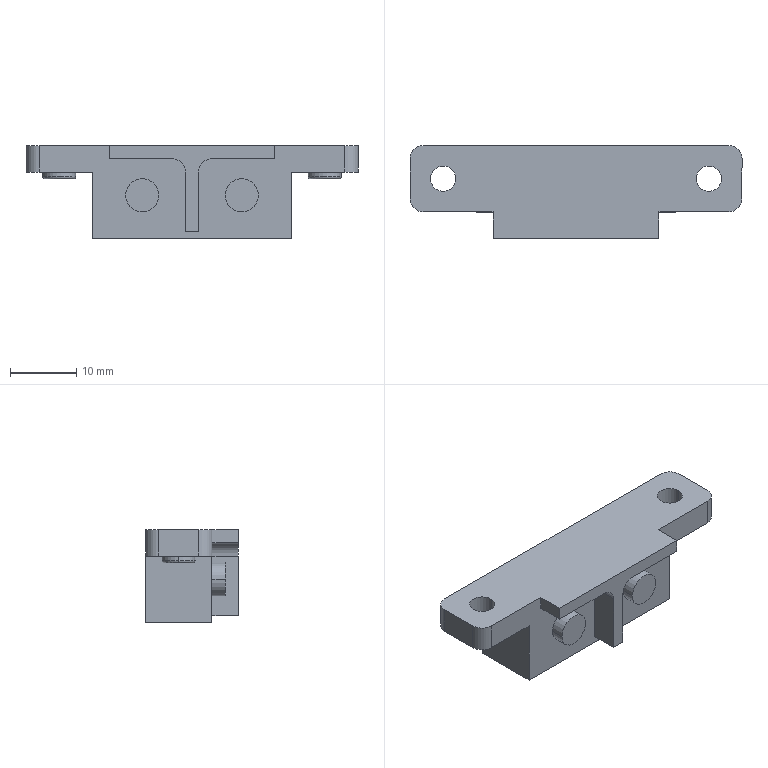Component | SolidWorks | SYM0671-81-200-1_SYMA1-51-omr_gls-s1-1 | 1 solid | 46 faces | volume 5284 mm3 | plane 20 | cylinder 18 | torus 8 | commonest cylinder face diameters 5 x8 4 x6 3.8 x4 | material ﾃﾞﾙﾘﾝ